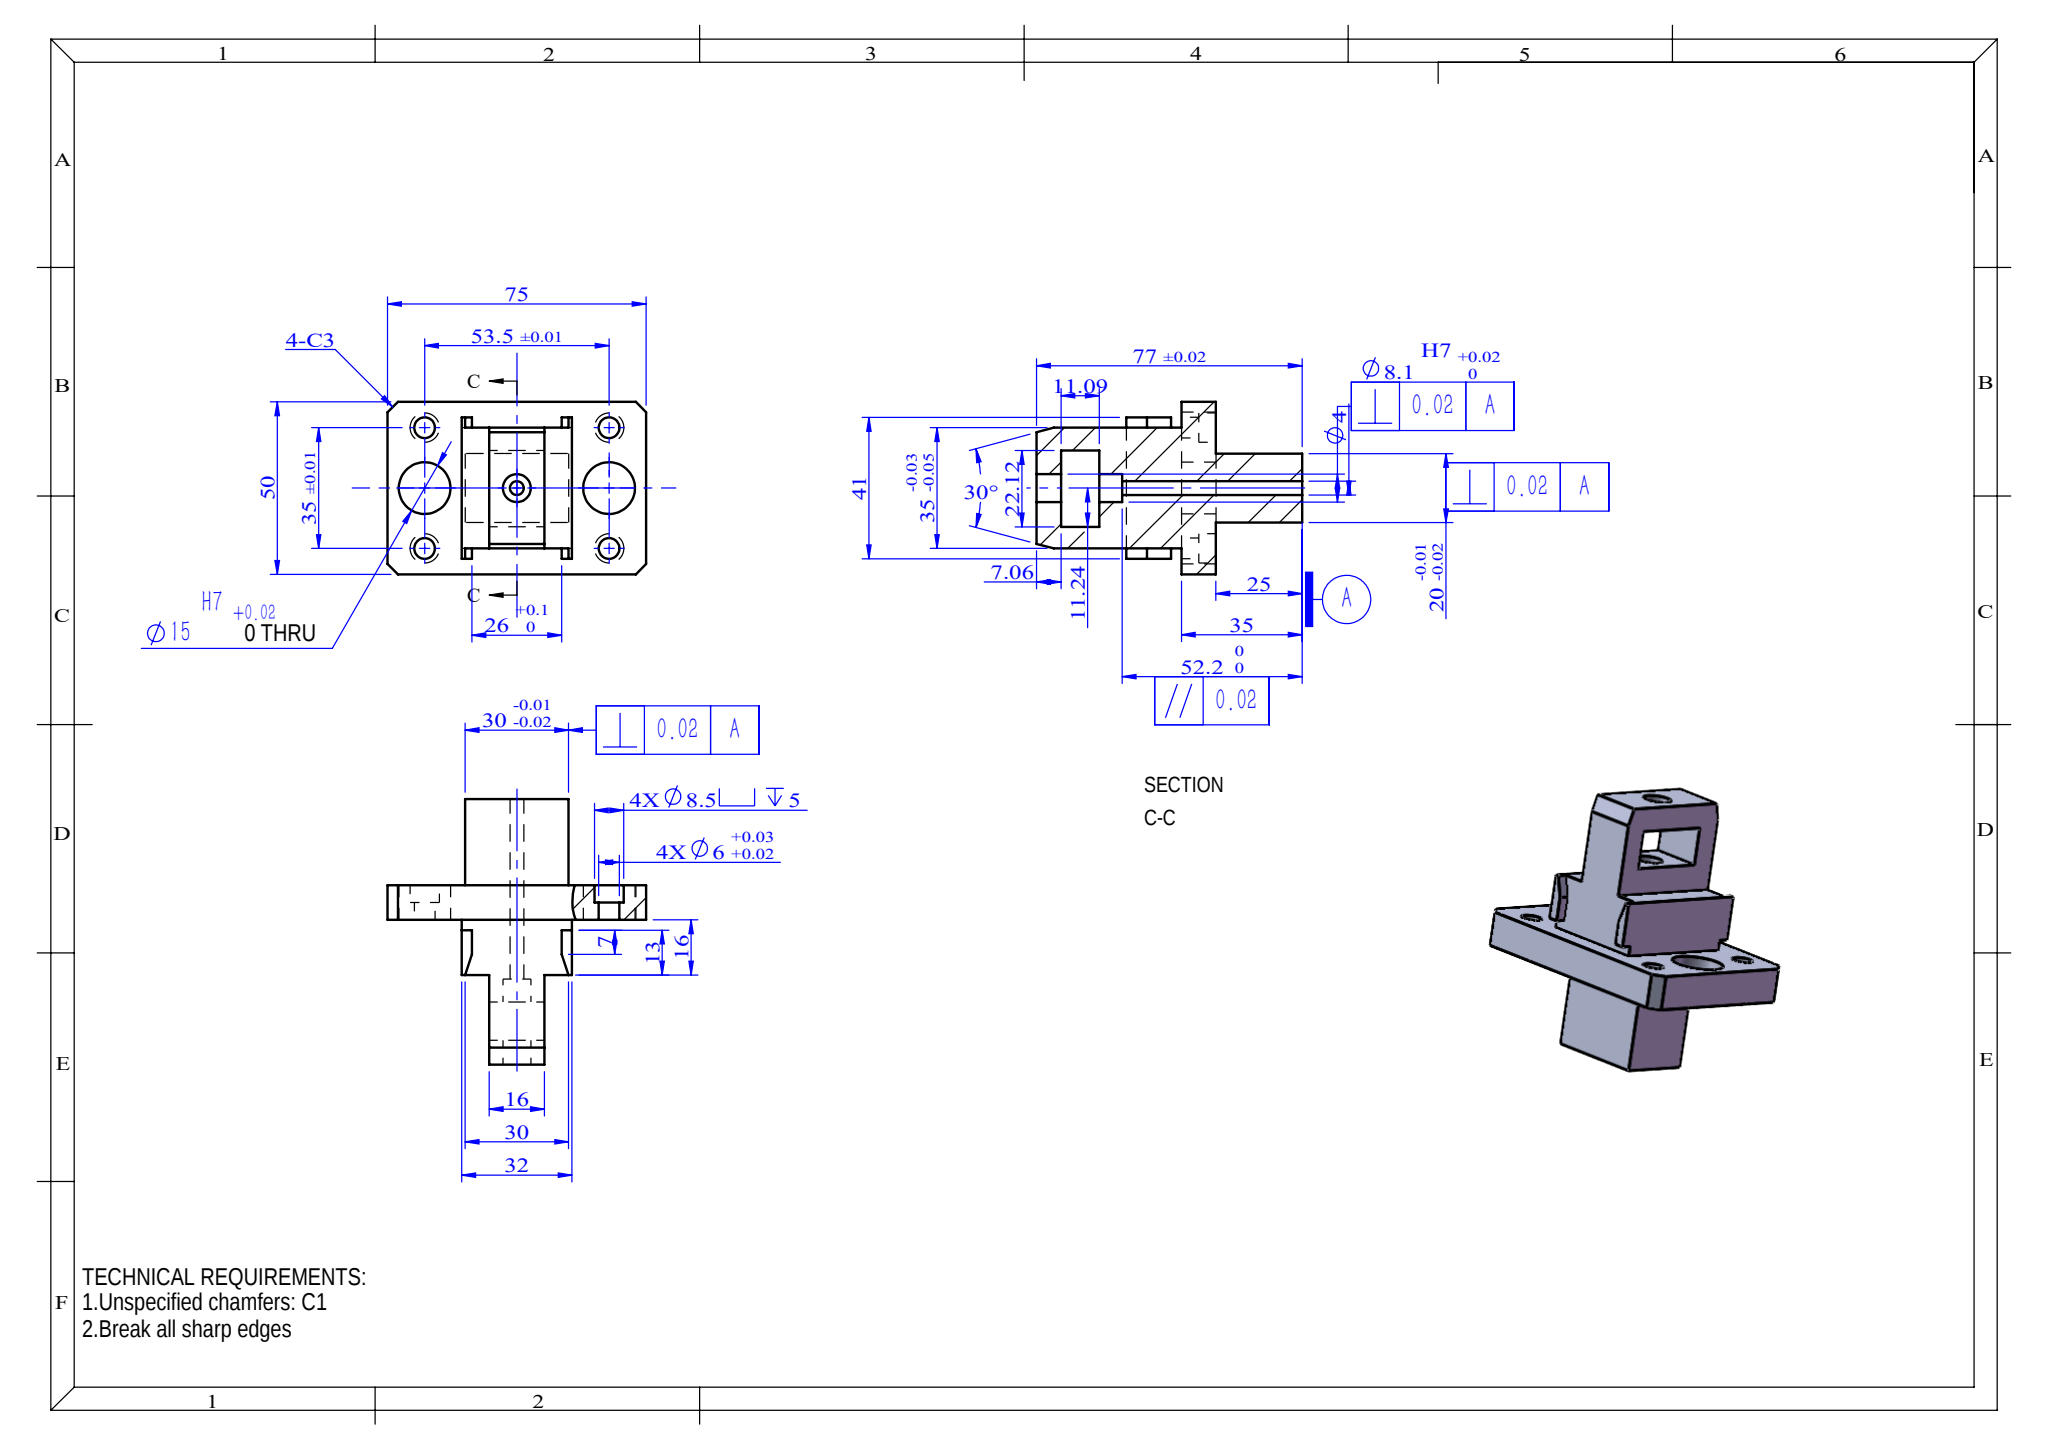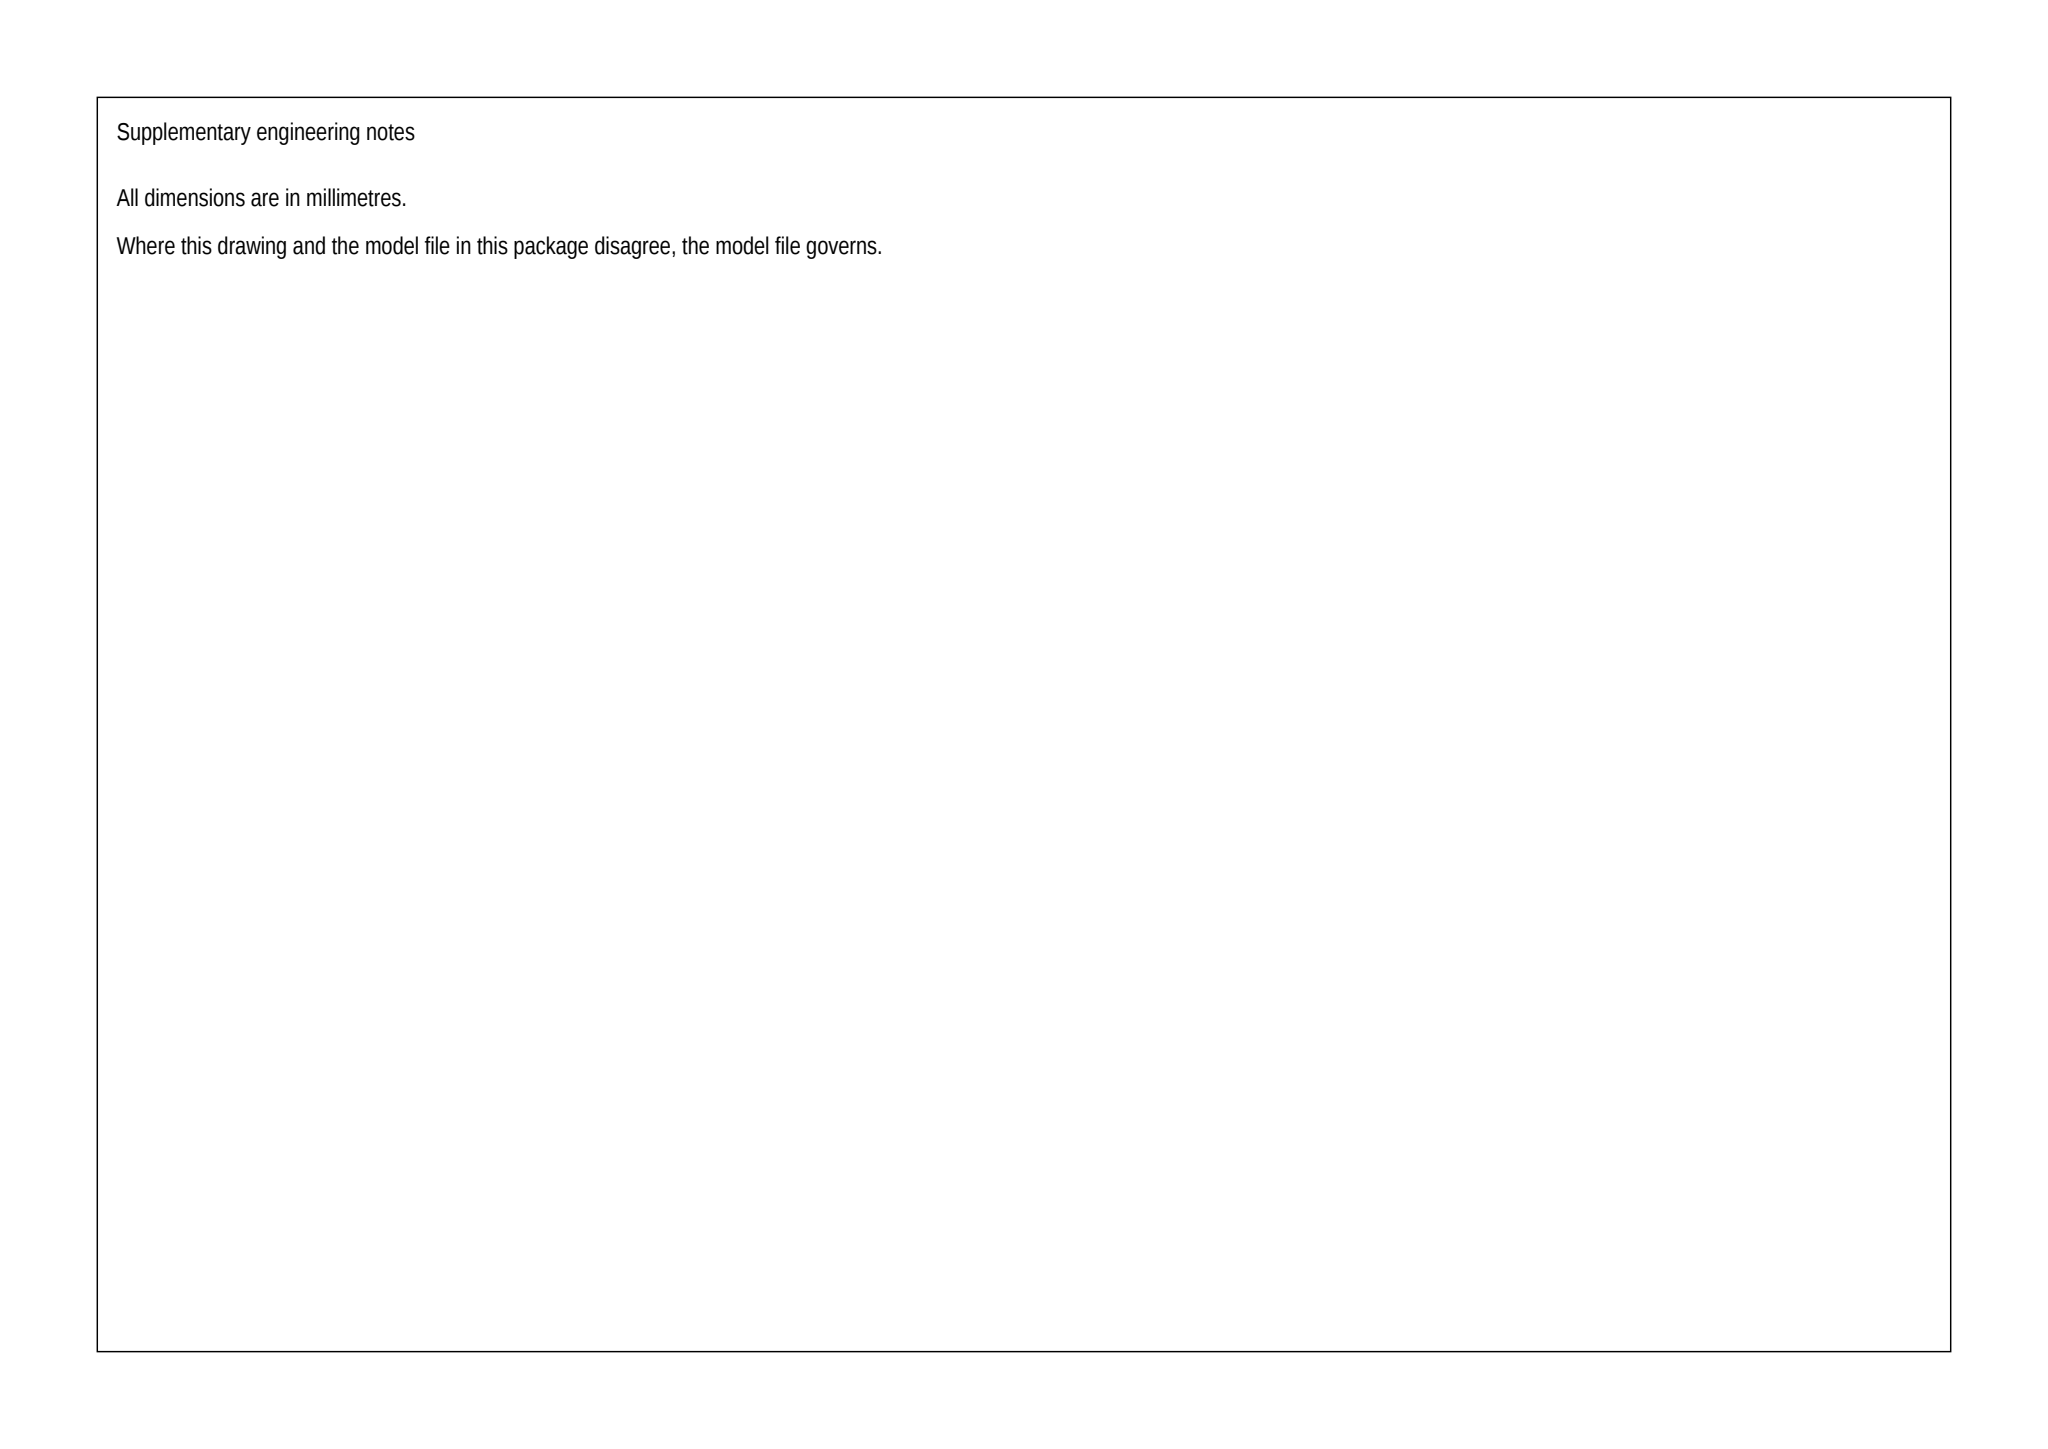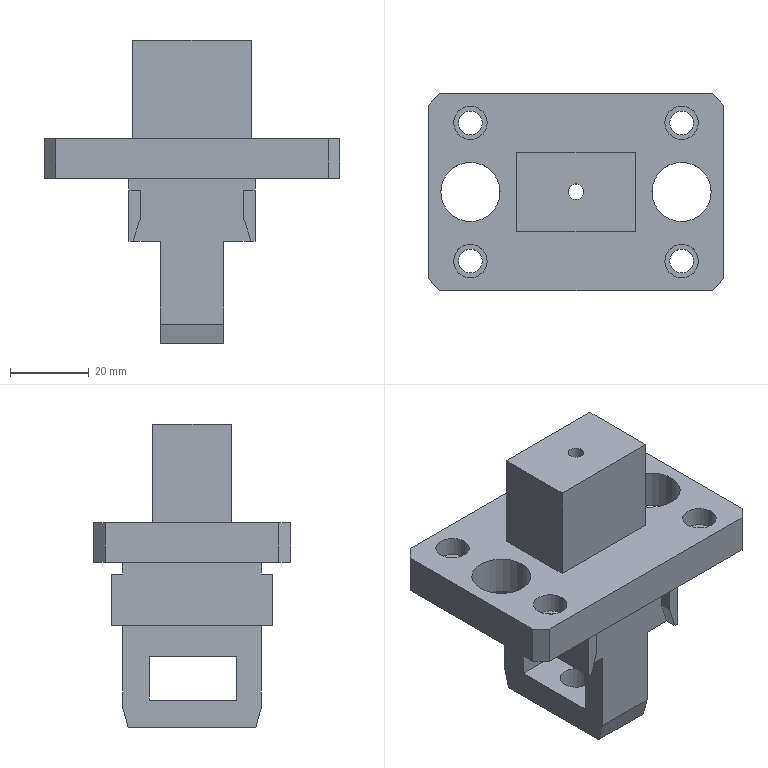Part | SolidWorks | mm | 1 solid | 77 faces | box 75 x 50 x 77 mm | volume 74568 mm3 | plane 51 | cylinder 26 | commonest cylinder face diameters 8.5 x8 6 x8 8.1 x4 15 x4 4 x2
Drawing notes:
ALL DIMENSIONS ARE IN MILLIMETERS (mm) UNLESS OTHERWISE STATED. | from the solid: STEP model units: mm (bbox_xyz 75.0 x 50.0 x 77.0 mm)
Upper boss angled face: bevel at 30° to the boss side face, located between Z=52.0 and Z=77.0 from the base-plate bottom face (datum A). | from the solid: axis_planes z = 52.0 and z = 77.0; bbox height 77.0
Lower boss / base-plate transition faces lie at Z=26.0 and Z=39.0 from the base-plate bottom face (datum A). | from the solid: axis_planes z = 26.0 (count 2) and z = 39.0 (count 4)
ALL DIMENSIONS ARE IN MILLIMETERS (mm) UNLESS OTHERWISE SPECIFIED. | from the solid: STEP model facts stated in mm; bbox_xyz = [75.0, 50.0, 77.0] mm
4X Ø6 +0.03/+0.02 BLIND, DP 5 BELOW Ø8.5 CBORE DP 5 (NOT THRU); HOLES AT X=10.75 & 64.25, Y=7.5 & 42.5 FROM BBOX MIN CORNER, I.E. 53.5 x 35 BOLT PATTERN ON PLATE TOP FACE Z=47 FROM DATUM A | from the solid: cylinders [6.0,'z',[10.75/64.25, 7.5/42.5],5.0] with mating [8.5,'z',same centres,5.0]; z plane at 47.0
2X Ø15 H7 (+0.02/0) THRU BASE PLATE, Z=42 TO 52 FROM DATUM A; HOLE AXES ON PLATE CENTRELINE Y=25, AT X=10.75 AND X=64.25 FROM BBOX MIN CORNER (53.5 APART, SYMMETRIC ABOUT PLATE CENTRE) | from the solid: cylinders: 2X dia 15.0 z-axis at [10.8,25.0] and [64.3,25.0], from 42.0 to 52.0
Ø8.1 H7 BORE ON AXIS X=37.5, Y=25: LOWER SEGMENT Z=0 TO 7.06 AND UPPER SEGMENT Z=18.15 TO 24.8 FROM DATUM A | from the solid: cylinders: dia 8.1 z-axis at [37.5,25.0] from 0.0 to 7.1 and from 18.1 to 24.8
Ø4 BORE ON SAME AXIS X=37.5, Y=25, FROM Z=24.8 THRU TO Z=77.0 (TOP OF UPPER BOSS) | from the solid: cylinders: dia 4.0 z-axis at [37.5,25.0] from 24.8 to 77.0
RECTANGULAR THRU OPENING IN LOWER BOSS: 22.1 WIDE (Y=13.8 TO 35.9) X 11.09 HIGH (Z=7.06 TO 18.15 FROM DATUM A), THROUGH BOSS IN X FROM X=29.5 TO X=45.5 | from the solid: axis_planes: y=13.8 and y=35.9 extents x[29.5,45.5] z[7.1,18.1]; z=7.1 and z=18.1 extents x[29.5,45.5] y[13.8,35.9]
LOWER BOSS TAPERED TRANSITION: 2X SIDE FACE AT 15° TO THE BOSS SIDE FACE, FROM Z=0 TO Z=5 FROM DATUM A; Y WIDTH 32.4 (Y=8.8 TO 41.2) AT Z=0 OPENING TO 35 (Y=7.5 TO 42.5) AT Z=5 | from the solid: inclined_planes: angle_to_xyz [90.0,15.0,75.0], bbox_from [29.5,41.2,0.0] and [29.5,7.5,0.0], size [16.0,1.3,5.0]; plane z=0 extent y[8.8,41.2]
4X LOWER-BOSS / BASE-PLATE TRANSITION FACE INCLINED 18.4° TO Z, EACH 2 (X) X 3 (Y) X 6 (Z), STARTING AT X=22.5 AND X=50.5, Y=4.5 AND Y=42.5, Z=26 FROM DATUM A | from the solid: inclined_planes: 4X angle_to_xyz [18.4,90.0,71.6], bbox_from [22.5/50.5, 4.5/42.5, 26.0], size [2.0,3.0,6.0]
build123d program:
from build123d import *

# Parameters (mm, degrees)
SKETCH1_W                = 32
SKETCH1_H                = 35
BOSS_EXTRUDE1_DEPTH      = 42
SKETCH2_W                = 75
SKETCH2_H                = 50
BOSS_EXTRUDE2_DEPTH      = 10
SKETCH3_W                = 30
SKETCH3_H                = 20
BOSS_EXTRUDE3_DEPTH      = 25
SKETCH4_R                = 7.5
CUT_EXTRUDE1_DEPTH       = 81.203
SKETCH5_R                = 4.05
CUT_EXTRUDE2_DEPTH       = 24.8
SKETCH6_W                = 3
SKETCH6_H                = 13
BOSS_EXTRUDE4_DEPTH      = 3
CHAMFER2_SIZE            = 5
CHAMFER2_SIZE2           = 1.34
CHAMFER3_SIZE            = 5
CHAMFER3_SIZE2           = 1.34
SKETCH9_W                = 8
SKETCH9_H                = 26
CUT_EXTRUDE5_DEPTH       = 103.944
CUT_EXTRUDE6_DEPTH       = 3
F_6_0_6_DIAMETER_HOLE1_D = 6
SKETCH13_R               = 4.25
CUT_EXTRUDE7_DEPTH       = 5
CHAMFER4_SIZE            = 3
SKETCH15_R               = 2
CUT_EXTRUDE8_DEPTH       = 86.985
SKETCH16_W               = 11.089
SKETCH16_H               = 22.117
CUT_EXTRUDE9_DEPTH       = 56


with BuildPart() as part:
    # Sketch1 → Boss-Extrude1 (new body)
    with BuildSketch(Plane.XY):
        with Locations((16, 17.5)):
            Rectangle(SKETCH1_W, SKETCH1_H)
    extrude(amount=BOSS_EXTRUDE1_DEPTH)

    # Sketch2 → Boss-Extrude2 (add)
    with BuildSketch(Plane.XY.offset(42)):
        with Locations((16, 17.5)):
            Rectangle(SKETCH2_W, SKETCH2_H)
    extrude(amount=BOSS_EXTRUDE2_DEPTH)

    # Sketch3 → Boss-Extrude3 (add)
    with BuildSketch(Plane.XY.offset(52)):
        with Locations((16, 17.5)):
            Rectangle(SKETCH3_W, SKETCH3_H)
    extrude(amount=BOSS_EXTRUDE3_DEPTH)

    # Sketch4 → Cut-Extrude1 (cut, through all)
    with BuildSketch(Plane(origin=(0, 0, 42), x_dir=(-1, 0, 0), z_dir=(0, 0, -1))):
        with Locations((-42.75, 17.5)):
            Circle(SKETCH4_R)
        with Locations(Location((10.75, 17.5, 0), (0, 0, 180))):
            Circle(SKETCH4_R)
    extrude(amount=-CUT_EXTRUDE1_DEPTH, mode=Mode.SUBTRACT)

    # Sketch5 → Cut-Extrude2 (cut)
    with BuildSketch(Plane(origin=(0, 0, 0), x_dir=(-1, 0, 0), z_dir=(0, 0, -1))):
        with Locations((-16, 17.5)):
            Circle(SKETCH5_R)
    extrude(amount=-CUT_EXTRUDE2_DEPTH, mode=Mode.SUBTRACT)

    # Sketch6 → Boss-Extrude4 (add)
    with BuildSketch(Plane(origin=(0, 0, 0), x_dir=(-1, 0, 0), z_dir=(0, -1, 0))):
        with Locations((-30.5, -32.5)):
            Rectangle(SKETCH6_W, SKETCH6_H)
        with Locations((-1.5, -32.5)):
            Rectangle(SKETCH6_W, SKETCH6_H)
    boss_extrude4 = extrude(amount=BOSS_EXTRUDE4_DEPTH)

    # Chamfer2
    chamfer2_edges = [part.edges().sort_by_distance(p)[0] for p in [
        (16, 35, 0),
    ]]
    chamfer2_side = [part.faces().sort_by_distance(p)[0] for p in [
        (16, 35, 21),
    ]]
    chamfer(chamfer2_edges, length=CHAMFER2_SIZE, length2=CHAMFER2_SIZE2, reference=chamfer2_side[0])

    # Chamfer3
    chamfer3_edges = [part.edges().sort_by_distance(p)[0] for p in [
        (16, 0, 0),
    ]]
    chamfer3_side = [part.faces().sort_by_distance(p)[0] for p in [
        (16, 0, 20.291),
    ]]
    chamfer(chamfer3_edges, length=CHAMFER3_SIZE, length2=CHAMFER3_SIZE2, reference=chamfer3_side[0])

    # Sketch9 → Cut-Extrude5 (cut, through all)
    with BuildSketch(Plane(origin=(0, 35, 0), x_dir=(1, 0, 0), z_dir=(0, 1, 0))):
        with Locations((4, -13)):
            Rectangle(SKETCH9_W, SKETCH9_H)
        with Locations((28, -13)):
            Rectangle(SKETCH9_W, SKETCH9_H)
    extrude(amount=-CUT_EXTRUDE5_DEPTH, mode=Mode.SUBTRACT)

    # Sketch10 → Cut-Extrude6 (cut)
    with BuildSketch(Plane(origin=(0, -3, 0), x_dir=(-1, 0, 0), z_dir=(0, -1, 0))):
        Polygon((-31, -26), (-29, -32), (-29, -26), align=None)
        Polygon((-3, -26), (-3, -32), (-1, -26), align=None)
    cut_extrude6 = extrude(amount=-CUT_EXTRUDE6_DEPTH, mode=Mode.SUBTRACT)

    # 6.0 _6_ Diameter Hole1 (through all)
    with Locations(Plane(origin=(0, 0, 42), x_dir=(-1, 0, 0), z_dir=(0, 0, -1))):
        with Locations((-42.75, 0), (-42.75, 35)):
            f_6_0_6_diameter_hole1 = Hole(F_6_0_6_DIAMETER_HOLE1_D / 2)

    # Sketch13 → Cut-Extrude7 (cut)
    with BuildSketch(Plane.XY.offset(52)):
        with Locations((42.75, 0)):
            Circle(SKETCH13_R)
        with Locations((42.75, 35)):
            Circle(SKETCH13_R)
    cut_extrude7 = extrude(amount=-CUT_EXTRUDE7_DEPTH, mode=Mode.SUBTRACT)

    # Chamfer4
    chamfer4_edges = [part.edges().sort_by_distance(p)[0] for p in [
        (-21.5, 42.5, 47),
        (-21.5, -7.5, 47),
        (53.5, -7.5, 47),
        (53.5, 42.5, 47),
    ]]
    chamfer(chamfer4_edges, length=CHAMFER4_SIZE)

    # Mirror17: 6.0 _6_ Diameter Hole1, Cut-Extrude7 across plane
    add(f_6_0_6_diameter_hole1.mirror(Plane(origin=(16, 0, 0), x_dir=(0, 0, 1), z_dir=(1, 0, 0))), mode=Mode.SUBTRACT)
    add(cut_extrude7.mirror(Plane(origin=(16, 0, 0), x_dir=(0, 0, 1), z_dir=(1, 0, 0))), mode=Mode.SUBTRACT)

    # Sketch15 → Cut-Extrude8 (cut, through all)
    with BuildSketch(Plane(origin=(0, 0, 24.8), x_dir=(-1, 0, 0), z_dir=(0, 0, -1))):
        with Locations((-16, 17.5)):
            Circle(SKETCH15_R)
    extrude(amount=-CUT_EXTRUDE8_DEPTH, mode=Mode.SUBTRACT)

    # Mirror18: Boss-Extrude4, Cut-Extrude6 across plane
    add(boss_extrude4.mirror(Plane.ZX.offset(17.5)))
    add(cut_extrude6.mirror(Plane.ZX.offset(17.5)), mode=Mode.SUBTRACT)

    # Sketch16 → Cut-Extrude9 (cut)
    with BuildSketch(Plane.ZY.offset(-8)):
        with Locations((12.606, 17.317)):
            Rectangle(SKETCH16_W, SKETCH16_H)
    extrude(amount=-CUT_EXTRUDE9_DEPTH, mode=Mode.SUBTRACT)


solid = part.part